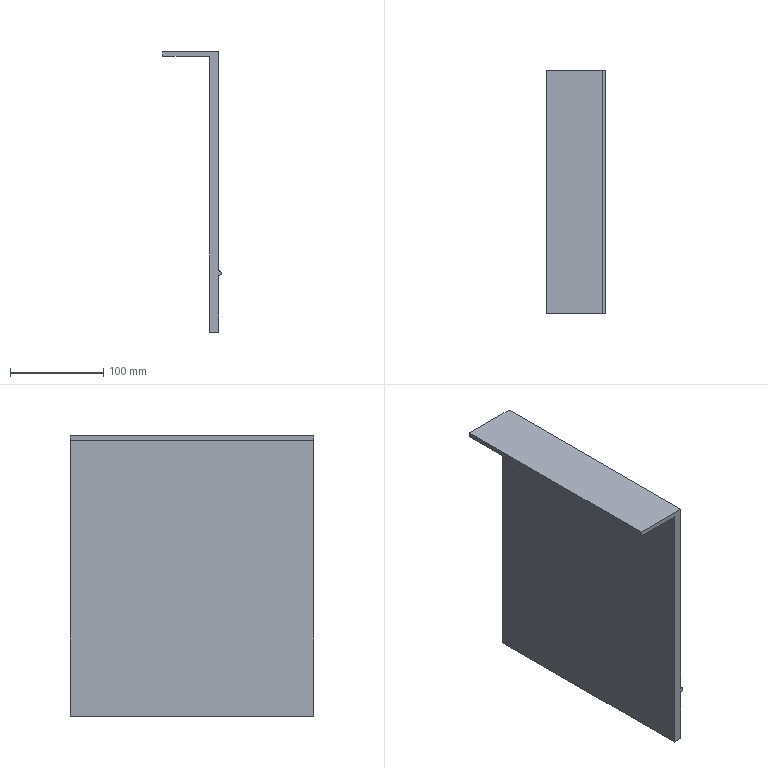Component | SolidWorks | TrackPlate-1 | 1 solid | 10 faces | box 62.5 x 260 x 300 mm | volume 847553 mm3 | plane 9 | cylinder 1 | commonest cylinder face diameters 5 x1
build123d program:
from build123d import *

# Parameters (mm, degrees)
SKETCH1_W           = 60
SKETCH1_H           = 260
BOSS_EXTRUDE1_DEPTH = 5
SKETCH2_W           = 300
SKETCH2_H           = 260
BOSS_EXTRUDE2_DEPTH = 10
SKETCH3_R           = 2.5
BOSS_EXTRUDE3_DEPTH = 260


with BuildPart() as part:
    # Sketch1 → Boss-Extrude1 (new body)
    with BuildSketch(Plane.XY):
        Rectangle(SKETCH1_W, SKETCH1_H)
    extrude(amount=BOSS_EXTRUDE1_DEPTH)

    # Sketch2 → Boss-Extrude2 (add)
    with BuildSketch(Plane.ZY.offset(30)):
        with Locations((150, 0)):
            Rectangle(SKETCH2_W, SKETCH2_H)
    extrude(amount=-BOSS_EXTRUDE2_DEPTH)

    # Sketch3 → Boss-Extrude3 (add)
    with BuildSketch(Plane(origin=(0, -130, 0), x_dir=(-1, 0, 0), z_dir=(0, -1, 0))):
        with Locations((30, -236.839)):
            Circle(SKETCH3_R)
    extrude(amount=-BOSS_EXTRUDE3_DEPTH)


solid = part.part

# Placed as in the assembly
solid = solid.moved(Location((-294.371, -1207.9, 415), (-180, 0, 180)))
STEP:
#1=COLOUR_RGB('',0.7922,0.8196,0.9333);
#2=FILL_AREA_STYLE_COLOUR('',#1);
#3=FILL_AREA_STYLE('',(#2));
#4=SURFACE_STYLE_FILL_AREA(#3);
#5=SURFACE_SIDE_STYLE('',(#4));
#6=SURFACE_STYLE_USAGE(.BOTH.,#5);
#7=PRESENTATION_STYLE_ASSIGNMENT((#6));
#8=CARTESIAN_POINT('',(-10.408,-42.437,4.528));
#9=VERTEX_POINT('',#8);
#10=CARTESIAN_POINT('',(-10.408,-42.437,6.916));
#11=VERTEX_POINT('',#10);
#12=CARTESIAN_POINT('',(-10.408,-42.437,16.142));
#13=DIRECTION('',(0.,-0.,1.));
#14=VECTOR('',#13,39.37);
#15=LINE('',#12,#14);
#16=EDGE_CURVE('',#9,#11,#15,.T.);
#17=ORIENTED_EDGE('',*,*,#16,.T.);
#18=CARTESIAN_POINT('',(-10.408,-52.673,6.916));
#19=VERTEX_POINT('',#18);
#20=CARTESIAN_POINT('',(-10.408,-42.159,6.916));
#21=DIRECTION('',(0.,-1.,-0.));
#22=VECTOR('',#21,39.37);
#23=LINE('',#20,#22);
#24=EDGE_CURVE('',#11,#19,#23,.T.);
#25=ORIENTED_EDGE('',*,*,#24,.T.);
#26=CARTESIAN_POINT('',(-10.408,-52.673,4.528));
#27=VERTEX_POINT('',#26);
#28=CARTESIAN_POINT('',(-10.408,-52.673,16.142));
#29=DIRECTION('',(0.,-0.,1.));
#30=VECTOR('',#29,39.37);
#31=LINE('',#28,#30);
#32=EDGE_CURVE('',#27,#19,#31,.T.);
#33=ORIENTED_EDGE('',*,*,#32,.F.);
#34=CARTESIAN_POINT('',(-10.408,-42.437,4.528));
#35=DIRECTION('',(-0.,1.,0.));
#36=VECTOR('',#35,39.37);
#37=LINE('',#34,#36);
#38=EDGE_CURVE('',#27,#9,#37,.T.);
#39=ORIENTED_EDGE('',*,*,#38,.T.);
#40=EDGE_LOOP('',(#17,#25,#33,#39));
#41=FACE_OUTER_BOUND('',#40,.T.);
#42=CARTESIAN_POINT('',(-10.408,-52.673,16.142));
#43=DIRECTION('',(-1.,-0.,0.));
#44=DIRECTION('',(0.,-0.,1.));
#45=AXIS2_PLACEMENT_3D('',#42,#43,#44);
#46=PLANE('',#45);
#47=ADVANCED_FACE('',(#41),#46,.F.);
#48=CARTESIAN_POINT('',(-10.802,-52.673,16.142));
#49=VERTEX_POINT('',#48);
#50=CARTESIAN_POINT('',(-10.802,-42.437,16.142));
#51=VERTEX_POINT('',#50);
#52=CARTESIAN_POINT('',(-10.802,-47.555,16.142));
#53=DIRECTION('',(-0.,1.,0.));
#54=VECTOR('',#53,39.37);
#55=LINE('',#52,#54);
#56=EDGE_CURVE('',#49,#51,#55,.T.);
#57=ORIENTED_EDGE('',*,*,#56,.F.);
#58=CARTESIAN_POINT('',(-12.77,-52.673,16.142));
#59=VERTEX_POINT('',#58);
#60=CARTESIAN_POINT('',(-10.408,-52.673,16.142));
#61=DIRECTION('',(-1.,-0.,0.));
#62=VECTOR('',#61,39.37);
#63=LINE('',#60,#62);
#64=EDGE_CURVE('',#49,#59,#63,.T.);
#65=ORIENTED_EDGE('',*,*,#64,.T.);
#66=CARTESIAN_POINT('',(-12.77,-42.437,16.142));
#67=VERTEX_POINT('',#66);
#68=CARTESIAN_POINT('',(-12.77,-52.673,16.142));
#69=DIRECTION('',(-0.,1.,0.));
#70=VECTOR('',#69,39.37);
#71=LINE('',#68,#70);
#72=EDGE_CURVE('',#59,#67,#71,.T.);
#73=ORIENTED_EDGE('',*,*,#72,.T.);
#74=CARTESIAN_POINT('',(-10.408,-42.437,16.142));
#75=DIRECTION('',(1.,0.,-0.));
#76=VECTOR('',#75,39.37);
#77=LINE('',#74,#76);
#78=EDGE_CURVE('',#67,#51,#77,.T.);
#79=ORIENTED_EDGE('',*,*,#78,.T.);
#80=EDGE_LOOP('',(#57,#65,#73,#79));
#81=FACE_OUTER_BOUND('',#80,.T.);
#82=CARTESIAN_POINT('',(-11.589,-47.555,16.142));
#83=DIRECTION('',(0.,-0.,1.));
#84=DIRECTION('',(1.,0.,-0.));
#85=AXIS2_PLACEMENT_3D('',#82,#83,#84);
#86=PLANE('',#85);
#87=ADVANCED_FACE('',(#81),#86,.F.);
#88=CARTESIAN_POINT('',(-12.77,-52.673,16.339));
#89=VERTEX_POINT('',#88);
#90=CARTESIAN_POINT('',(-12.77,-42.437,16.339));
#91=VERTEX_POINT('',#90);
#92=CARTESIAN_POINT('',(-12.77,-52.673,16.339));
#93=DIRECTION('',(-0.,1.,0.));
#94=VECTOR('',#93,39.37);
#95=LINE('',#92,#94);
#96=EDGE_CURVE('',#89,#91,#95,.T.);
#97=ORIENTED_EDGE('',*,*,#96,.T.);
#98=CARTESIAN_POINT('',(-12.77,-42.437,16.142));
#99=DIRECTION('',(0.,-0.,1.));
#100=VECTOR('',#99,39.37);
#101=LINE('',#98,#100);
#102=EDGE_CURVE('',#67,#91,#101,.T.);
#103=ORIENTED_EDGE('',*,*,#102,.F.);
#104=ORIENTED_EDGE('',*,*,#72,.F.);
#105=CARTESIAN_POINT('',(-12.77,-52.673,16.142));
#106=DIRECTION('',(0.,-0.,1.));
#107=VECTOR('',#106,39.37);
#108=LINE('',#105,#107);
#109=EDGE_CURVE('',#59,#89,#108,.T.);
#110=ORIENTED_EDGE('',*,*,#109,.T.);
#111=EDGE_LOOP('',(#97,#103,#104,#110));
#112=FACE_OUTER_BOUND('',#111,.T.);
#113=CARTESIAN_POINT('',(-12.77,-52.673,16.142));
#114=DIRECTION('',(1.,0.,-0.));
#115=DIRECTION('',(-0.,0.,-1.));
#116=AXIS2_PLACEMENT_3D('',#113,#114,#115);
#117=PLANE('',#116);
#118=ADVANCED_FACE('',(#112),#117,.F.);
#119=CARTESIAN_POINT('',(-10.408,-42.437,7.113));
#120=VERTEX_POINT('',#119);
#121=CARTESIAN_POINT('',(-10.408,-42.437,16.339));
#122=VERTEX_POINT('',#121);
#123=CARTESIAN_POINT('',(-10.408,-42.437,16.142));
#124=DIRECTION('',(0.,-0.,1.));
#125=VECTOR('',#124,39.37);
#126=LINE('',#123,#125);
#127=EDGE_CURVE('',#120,#122,#126,.T.);
#128=ORIENTED_EDGE('',*,*,#127,.F.);
#129=CARTESIAN_POINT('',(-10.408,-42.437,7.014));
#130=DIRECTION('',(-0.,1.,0.));
#131=DIRECTION('',(0.,0.,1.));
#132=AXIS2_PLACEMENT_3D('',#129,#130,#131);
#133=CIRCLE('',#132,0.09843);
#134=EDGE_CURVE('',#120,#11,#133,.T.);
#135=ORIENTED_EDGE('',*,*,#134,.T.);
#136=ORIENTED_EDGE('',*,*,#16,.F.);
#137=CARTESIAN_POINT('',(-10.802,-42.437,4.528));
#138=VERTEX_POINT('',#137);
#139=CARTESIAN_POINT('',(-10.802,-42.437,4.528));
#140=DIRECTION('',(1.,0.,-0.));
#141=VECTOR('',#140,39.37);
#142=LINE('',#139,#141);
#143=EDGE_CURVE('',#138,#9,#142,.T.);
#144=ORIENTED_EDGE('',*,*,#143,.F.);
#145=CARTESIAN_POINT('',(-10.802,-42.437,16.339));
#146=DIRECTION('',(0.,-0.,1.));
#147=VECTOR('',#146,39.37);
#148=LINE('',#145,#147);
#149=EDGE_CURVE('',#138,#51,#148,.T.);
#150=ORIENTED_EDGE('',*,*,#149,.T.);
#151=ORIENTED_EDGE('',*,*,#78,.F.);
#152=ORIENTED_EDGE('',*,*,#102,.T.);
#153=CARTESIAN_POINT('',(-10.408,-42.437,16.339));
#154=DIRECTION('',(1.,0.,-0.));
#155=VECTOR('',#154,39.37);
#156=LINE('',#153,#155);
#157=EDGE_CURVE('',#91,#122,#156,.T.);
#158=ORIENTED_EDGE('',*,*,#157,.T.);
#159=EDGE_LOOP('',(#128,#135,#136,#144,#150,#151,#152,#158));
#160=FACE_OUTER_BOUND('',#159,.T.);
#161=CARTESIAN_POINT('',(-10.408,-42.437,16.142));
#162=DIRECTION('',(0.,-1.,-0.));
#163=DIRECTION('',(0.,-0.,1.));
#164=AXIS2_PLACEMENT_3D('',#161,#162,#163);
#165=PLANE('',#164);
#166=ADVANCED_FACE('',(#160),#165,.F.);
#167=CARTESIAN_POINT('',(-10.408,-52.673,7.113));
#168=VERTEX_POINT('',#167);
#169=CARTESIAN_POINT('',(-10.408,-52.673,16.339));
#170=VERTEX_POINT('',#169);
#171=CARTESIAN_POINT('',(-10.408,-52.673,16.142));
#172=DIRECTION('',(0.,-0.,1.));
#173=VECTOR('',#172,39.37);
#174=LINE('',#171,#173);
#175=EDGE_CURVE('',#168,#170,#174,.T.);
#176=ORIENTED_EDGE('',*,*,#175,.F.);
#177=CARTESIAN_POINT('',(-10.408,-42.159,7.113));
#178=DIRECTION('',(-0.,1.,0.));
#179=VECTOR('',#178,39.37);
#180=LINE('',#177,#179);
#181=EDGE_CURVE('',#168,#120,#180,.T.);
#182=ORIENTED_EDGE('',*,*,#181,.T.);
#183=ORIENTED_EDGE('',*,*,#127,.T.);
#184=CARTESIAN_POINT('',(-10.408,-52.673,16.339));
#185=DIRECTION('',(0.,-1.,-0.));
#186=VECTOR('',#185,39.37);
#187=LINE('',#184,#186);
#188=EDGE_CURVE('',#122,#170,#187,.T.);
#189=ORIENTED_EDGE('',*,*,#188,.T.);
#190=EDGE_LOOP('',(#176,#182,#183,#189));
#191=FACE_OUTER_BOUND('',#190,.T.);
#192=CARTESIAN_POINT('',(-10.408,-52.673,16.142));
#193=DIRECTION('',(-1.,-0.,0.));
#194=DIRECTION('',(0.,-0.,1.));
#195=AXIS2_PLACEMENT_3D('',#192,#193,#194);
#196=PLANE('',#195);
#197=ADVANCED_FACE('',(#191),#196,.F.);
#198=ORIENTED_EDGE('',*,*,#32,.T.);
#199=CARTESIAN_POINT('',(-10.408,-52.673,7.014));
#200=DIRECTION('',(0.,-1.,-0.));
#201=DIRECTION('',(0.,0.,1.));
#202=AXIS2_PLACEMENT_3D('',#199,#200,#201);
#203=CIRCLE('',#202,0.09843);
#204=EDGE_CURVE('',#19,#168,#203,.T.);
#205=ORIENTED_EDGE('',*,*,#204,.T.);
#206=ORIENTED_EDGE('',*,*,#175,.T.);
#207=CARTESIAN_POINT('',(-10.408,-52.673,16.339));
#208=DIRECTION('',(-1.,-0.,0.));
#209=VECTOR('',#208,39.37);
#210=LINE('',#207,#209);
#211=EDGE_CURVE('',#170,#89,#210,.T.);
#212=ORIENTED_EDGE('',*,*,#211,.T.);
#213=ORIENTED_EDGE('',*,*,#109,.F.);
#214=ORIENTED_EDGE('',*,*,#64,.F.);
#215=CARTESIAN_POINT('',(-10.802,-52.673,4.528));
#216=VERTEX_POINT('',#215);
#217=CARTESIAN_POINT('',(-10.802,-52.673,16.339));
#218=DIRECTION('',(-0.,0.,-1.));
#219=VECTOR('',#218,39.37);
#220=LINE('',#217,#219);
#221=EDGE_CURVE('',#49,#216,#220,.T.);
#222=ORIENTED_EDGE('',*,*,#221,.T.);
#223=CARTESIAN_POINT('',(-10.802,-52.673,4.528));
#224=DIRECTION('',(1.,0.,-0.));
#225=VECTOR('',#224,39.37);
#226=LINE('',#223,#225);
#227=EDGE_CURVE('',#216,#27,#226,.T.);
#228=ORIENTED_EDGE('',*,*,#227,.T.);
#229=EDGE_LOOP('',(#198,#205,#206,#212,#213,#214,#222,#228));
#230=FACE_OUTER_BOUND('',#229,.T.);
#231=CARTESIAN_POINT('',(-10.408,-52.673,16.142));
#232=DIRECTION('',(-0.,1.,0.));
#233=DIRECTION('',(-0.,0.,-1.));
#234=AXIS2_PLACEMENT_3D('',#231,#232,#233);
#235=PLANE('',#234);
#236=ADVANCED_FACE('',(#230),#235,.F.);
#237=ORIENTED_EDGE('',*,*,#188,.F.);
#238=ORIENTED_EDGE('',*,*,#157,.F.);
#239=ORIENTED_EDGE('',*,*,#96,.F.);
#240=ORIENTED_EDGE('',*,*,#211,.F.);
#241=EDGE_LOOP('',(#237,#238,#239,#240));
#242=FACE_OUTER_BOUND('',#241,.T.);
#243=CARTESIAN_POINT('',(-11.589,-47.555,16.339));
#244=DIRECTION('',(0.,-0.,1.));
#245=DIRECTION('',(1.,0.,-0.));
#246=AXIS2_PLACEMENT_3D('',#243,#244,#245);
#247=PLANE('',#246);
#248=ADVANCED_FACE('',(#242),#247,.T.);
#249=ORIENTED_EDGE('',*,*,#221,.F.);
#250=ORIENTED_EDGE('',*,*,#56,.T.);
#251=ORIENTED_EDGE('',*,*,#149,.F.);
#252=CARTESIAN_POINT('',(-10.802,-42.437,4.528));
#253=DIRECTION('',(-0.,1.,0.));
#254=VECTOR('',#253,39.37);
#255=LINE('',#252,#254);
#256=EDGE_CURVE('',#216,#138,#255,.T.);
#257=ORIENTED_EDGE('',*,*,#256,.F.);
#258=EDGE_LOOP('',(#249,#250,#251,#257));
#259=FACE_OUTER_BOUND('',#258,.T.);
#260=CARTESIAN_POINT('',(-10.802,-47.555,16.339));
#261=DIRECTION('',(1.,0.,-0.));
#262=DIRECTION('',(-0.,0.,-1.));
#263=AXIS2_PLACEMENT_3D('',#260,#261,#262);
#264=PLANE('',#263);
#265=ADVANCED_FACE('',(#259),#264,.F.);
#266=ORIENTED_EDGE('',*,*,#38,.F.);
#267=ORIENTED_EDGE('',*,*,#227,.F.);
#268=ORIENTED_EDGE('',*,*,#256,.T.);
#269=ORIENTED_EDGE('',*,*,#143,.T.);
#270=EDGE_LOOP('',(#266,#267,#268,#269));
#271=FACE_OUTER_BOUND('',#270,.T.);
#272=CARTESIAN_POINT('',(-10.802,-42.437,4.528));
#273=DIRECTION('',(-0.,0.,-1.));
#274=DIRECTION('',(0.,-1.,-0.));
#275=AXIS2_PLACEMENT_3D('',#272,#273,#274);
#276=PLANE('',#275);
#277=ADVANCED_FACE('',(#271),#276,.T.);
#278=ORIENTED_EDGE('',*,*,#24,.F.);
#279=ORIENTED_EDGE('',*,*,#134,.F.);
#280=ORIENTED_EDGE('',*,*,#181,.F.);
#281=ORIENTED_EDGE('',*,*,#204,.F.);
#282=EDGE_LOOP('',(#278,#279,#280,#281));
#283=FACE_OUTER_BOUND('',#282,.T.);
#284=CARTESIAN_POINT('',(-10.408,-42.159,7.014));
#285=DIRECTION('',(0.,-1.,-0.));
#286=DIRECTION('',(0.,0.,1.));
#287=AXIS2_PLACEMENT_3D('',#284,#285,#286);
#288=CYLINDRICAL_SURFACE('',#287,0.09843);
#289=ADVANCED_FACE('',(#283),#288,.T.);
#290=CLOSED_SHELL('',(#47,#87,#118,#166,#197,#236,#248,#265,#277,#289));
#291=MANIFOLD_SOLID_BREP('',#290);
#292=STYLED_ITEM('',(#7),#291);
#293=(LENGTH_UNIT()NAMED_UNIT(*)SI_UNIT($,.METRE.));
#294=LENGTH_MEASURE_WITH_UNIT(LENGTH_MEASURE(0.0254),#293);
#295=DIMENSIONAL_EXPONENTS(1.,0.,0.,0.,0.,0.,0.);
#296=(CONVERSION_BASED_UNIT('',#294)LENGTH_UNIT()NAMED_UNIT(#295));
#297=UNCERTAINTY_MEASURE_WITH_UNIT(LENGTH_MEASURE(0.00001),#296,'','');
#298=(NAMED_UNIT(*)PLANE_ANGLE_UNIT()SI_UNIT($,.RADIAN.));
#299=(NAMED_UNIT(*)SI_UNIT($,.STERADIAN.)SOLID_ANGLE_UNIT());
#300=(GEOMETRIC_REPRESENTATION_CONTEXT(3)GLOBAL_UNCERTAINTY_ASSIGNED_CONTEXT((#297))GLOBAL_UNIT_ASSIGNED_CONTEXT((#296,#298,#299))REPRESENTATION_CONTEXT('',''));
#301=MECHANICAL_DESIGN_GEOMETRIC_PRESENTATION_REPRESENTATION('',(#292),#300);
#302=CARTESIAN_POINT('',(0.,0.,0.));
#303=DIRECTION('',(0.,0.,1.));
#304=DIRECTION('',(1.,0.,0.));
#305=AXIS2_PLACEMENT_3D('',#302,#303,#304);
#306=(LENGTH_UNIT()NAMED_UNIT(*)SI_UNIT($,.METRE.));
#307=LENGTH_MEASURE_WITH_UNIT(LENGTH_MEASURE(0.0254),#306);
#308=DIMENSIONAL_EXPONENTS(1.,0.,0.,0.,0.,0.,0.);
#309=(CONVERSION_BASED_UNIT('',#307)LENGTH_UNIT()NAMED_UNIT(#308));
#310=UNCERTAINTY_MEASURE_WITH_UNIT(LENGTH_MEASURE(0.00001),#309,'','');
#311=(NAMED_UNIT(*)PLANE_ANGLE_UNIT()SI_UNIT($,.RADIAN.));
#312=(NAMED_UNIT(*)SI_UNIT($,.STERADIAN.)SOLID_ANGLE_UNIT());
#313=(GEOMETRIC_REPRESENTATION_CONTEXT(3)GLOBAL_UNCERTAINTY_ASSIGNED_CONTEXT((#310))GLOBAL_UNIT_ASSIGNED_CONTEXT((#309,#311,#312))REPRESENTATION_CONTEXT('',''));
#314=ADVANCED_BREP_SHAPE_REPRESENTATION('',(#291,#305),#313);
#315=PRESENTATION_LAYER_ASSIGNMENT('','',(#292));